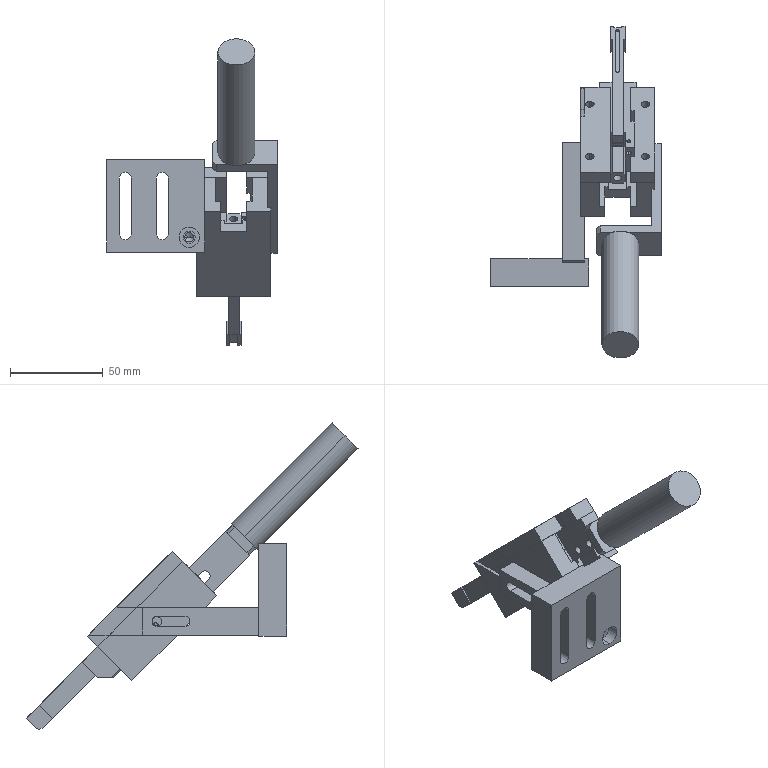Assembly | SolidWorks | mm | 12 component files | 12 solids | 233 faces | box 92 x 179.44 x 165.47 mm | volume 144263 mm3 | plane 140 | cylinder 71 | cone 22 | commonest cylinder face diameters 3 x16 3.3 x8 4.5 x8 4.2 x6 5.5 x5 6.5 x4 5 x4 2 x4
Bill of materials:
Cylinder16X30 | 1 |  | Plain solid round cylinder with flat ends, length roughly 2.5-3 times its diameter.
ZL-10-01BasePlate | 1 |  | Rectangular block or thick plate with two parallel obround through-slots, one round through-hole, and a shallow rectangular notch cut into one top edge.
ZL-10-02SupportPlate | 1 |  | Long rectangular bar with a round hole in one end face, chamfered edges around that end, and an obround through-slot near the opposite end of one side face.
ZL-10-03SlideChannel | 1 |  | Complex rectangular block with a stepped U-shaped slot open at one end, an open slot/channel at the other end, several stepped pockets, shallow side recesses, and four small holes in one face.
ZL-10-04LeftCoverPlate | 1 |  | Thin rectangular bar with two round holes along its length and a shallow rectangular notch or step on one long edge.
ZL-10-05RightCoverPlate | 1 |  | Thin rectangular bar with two round holes and a long shallow step/relief along one long edge between the holes, plus a short edge recess.
ZL-10-06L-shapedBracket | 1 |  | L-shaped angle bracket made from flat strip: the short leg has a round through-hole and chamfered end corners, and the long leg has an obround through-slot.
ZL-10-07Slider | 1 |  | Rectangular plate/block with a stepped open slot at one end, a narrower open slot at the other end, chamfered corners at one end, and several small holes on the faces and edges.
ZL-10-08FloatingJoint | 1 |  | Prismatic bar with a rectangular cross-section and chamfered long edges (octagon-like outline), with a round bore in each end face and a round cross-hole through a side face near one end.
ZL-10-10FloatingJointPin | 2 |  | Long solid round rod/pin with small chamfers at both ends, length roughly 6-7 times its diameter.
ZL3-10-09PressureBlock | 1 |  | Long slender flat strip with one rounded end holding a small round through-hole; near that end there are a small end notch and slightly wider shoulder/lug sections.
Mates:
1. concentric | ZL-10-01BasePlate-1 face at (18.823, -6.251, -17) dir (0, -1, 0) r 3.3 | ZL-10-02SupportPlate-1 face at (18.823, 6.749, -17) dir (0, -1, 0) r 2.5
2. coincident | ZL-10-01BasePlate-1 face at (12.823, 8.749, -25) dir (1, 0, 0) | ZL-10-02SupportPlate-1 face at (12.823, 71.749, -9.5) dir (-1, 0, 0)
3. coincident | ZL-10-01BasePlate-1 face at (24.823, 6.749, -25) dir (0, 1, 0) | ZL-10-02SupportPlate-1 face at (24.823, 6.749, -9.5) dir (0, -1, 0)
4. concentric | ZL-10-02SupportPlate-1 face at (12.823, 63.749, -17) dir (1, 0, 0) r 2.75 | ZL-10-03SlideChannel-1 face at (24.823, 63.749, -17) dir (-1, 0, 0) r 2.5
5. coincident | ZL-10-02SupportPlate-1 face at (24.823, 6.749, -24.5) dir (0, 0, -1) | ZL-10-03SlideChannel-1 face at (24.823, 89.634, -24.5) dir (0, 0, 1)
6. coincident | ZL-10-02SupportPlate-1 face at (24.823, 71.749, -9.5) dir (1, 0, 0) | ZL-10-03SlideChannel-1 face at (24.823, 74.634, -9.5) dir (-1, 0, 0)
7. concentric | ZL-10-03SlideChannel-1 face at (61.323, 52.007, -6.672) dir (1, 0, 0) r 2.1 | ZL-10-06L-shapedBracket-1 face at (31.323, 52.007, -6.672) dir (1, 0, 0) r 2.75
8. coincident | ZL-10-03SlideChannel-1 face at (61.323, 79.584, -46.977) dir (1, 0, 0) | ZL-10-06L-shapedBracket-1 face at (61.323, 13.823, 18.784) dir (-1, 0, 0)
9. coincident | ZL-10-03SlideChannel-1 face at (61.323, 92.312, -34.249) dir (0, -0.7071, -0.7071) | ZL-10-06L-shapedBracket-1 face at (66.323, 26.551, 31.512) dir (0, 0.7071, 0.7071)
10. coincident | ZL-10-03SlideChannel-1 plane at (42.823, 31.501, -3.136) dir (-1, 0, 0) | ZL-10-07Slider-1 plane at (42.823, 56.084, -16.405) dir (-1, 0, 0)
11. coincident | ZL-10-03SlideChannel-1 face at (52.823, 83.119, -43.441) dir (0, 0.7071, 0.7071) | ZL-10-07Slider-1 face at (32.823, 91.439, -51.761) dir (0, -0.7071, -0.7071)
12. concentric | ZL-10-07Slider-1 face at (52.823, 64.569, -19.234) dir (-1, 0, 0) r 1.5 | ZL-10-08FloatingJoint-1 face at (38.823, 64.569, -19.234) dir (1, 0, 0) r 1.5
13. coincident | ZL-10-07Slider-1 plane at (42.823, 56.084, -16.405) dir (-1, 0, 0) | ZL-10-08FloatingJoint-1 plane at (42.823, 52.548, -7.213) dir (1, 0, 0)
14. coincident | ZL-10-07Slider-1 face at (45.823, 97.096, -46.104) dir (0, 0.7071, 0.7071) | ZL-10-08FloatingJoint-1 face at (38.823, 69.519, -18.527) dir (0, 0.7071, 0.7071)
15. coincident | ZL-10-03SlideChannel-1 face at (22.823, 95.847, -30.713) dir (0, 0.7071, 0.7071) | ZL-10-04LeftCoverPlate-1 face at (22.823, 95.847, -30.713) dir (0, -0.7071, -0.7071)
16. coincident | ZL-10-03SlideChannel-1 face at (62.823, 95.847, -30.713) dir (0, 0.7071, 0.7071) | ZL-10-05RightCoverPlate-1 face at (49.823, 95.847, -30.713) dir (0, -0.7071, -0.7071)
17. concentric | ZL-10-07Slider-1 face at (32.823, 75.883, -17.82) dir (1, 0, 0) r 1.5 | ZL3-10-09PressureBlock-1 face at (38.823, 75.883, -17.82) dir (1, 0, 0) r 1.5
18. coincident | ZL-10-07Slider-1 plane at (42.823, 56.084, -16.405) dir (-1, 0, 0) | ZL3-10-09PressureBlock-1 plane at (42.823, 75.175, -10.041) dir (1, 0, 0)
19. coincident | ZL-10-07Slider-1 face at (45.823, 97.096, -46.104) dir (0, 0.7071, 0.7071) | ZL3-10-09PressureBlock-1 face at (45.823, 68.104, -17.112) dir (0, -0.7071, -0.7071)
20. concentric | ZL-10-07Slider-1 face at (52.823, 64.569, -19.234) dir (-1, 0, 0) r 1.5 | ZL-10-10FloatingJointPin-1 face at (32.823, 64.569, -19.234) dir (1, 0, 0) r 1.5
21. coincident | ZL-10-07Slider-1 face at (52.823, 91.439, -51.761) dir (1, 0, 0) | ZL-10-10FloatingJointPin-1 face at (52.823, 64.569, -19.234) dir (1, 0, 0)
22. concentric | ZL-10-07Slider-1 face at (32.823, 75.883, -17.82) dir (1, 0, 0) r 1.5 | ZL-10-10FloatingJointPin-2 face at (52.823, 75.883, -17.82) dir (-1, 0, 0) r 1.5
23. coincident | ZL-10-07Slider-1 face at (52.823, 91.439, -51.761) dir (1, 0, 0) | ZL-10-10FloatingJointPin-2 face at (52.823, 75.883, -17.82) dir (1, 0, 0)
24. concentric | ZL-10-03SlideChannel-1 face at (27.823, 58.371, 6.763) dir (0, 0.7071, 0.7071) r 1.65 | ZL-10-04LeftCoverPlate-1 face at (27.823, 58.371, 6.763) dir (0, 0.7071, 0.7071) r 2.25
25. concentric | ZL-10-03SlideChannel-1 face at (27.823, 86.655, -21.521) dir (0, 0.7071, 0.7071) r 1.65 | ZL-10-04LeftCoverPlate-1 face at (27.823, 86.655, -21.521) dir (0, 0.7071, 0.7071) r 2.25
26. concentric | ZL-10-03SlideChannel-1 face at (57.823, 86.655, -21.521) dir (0, 0.7071, 0.7071) r 1.65 | ZL-10-05RightCoverPlate-1 face at (57.823, 86.655, -21.521) dir (0, 0.7071, 0.7071) r 2.25
27. concentric | ZL-10-03SlideChannel-1 face at (57.823, 58.371, 6.763) dir (0, 0.7071, 0.7071) r 1.65 | ZL-10-05RightCoverPlate-1 face at (57.823, 58.371, 6.763) dir (0, 0.7071, 0.7071) r 2.25
28. concentric | ZL-10-06L-shapedBracket-1 face at (44.323, 66.149, -20.814) dir (0, -0.7071, 0.7071) r 5.25 | Cylinder16X30-1 face at (44.323, -37.796, 83.131) dir (0, 0.7071, -0.7071) r 10
29. coincident | ZL-10-06L-shapedBracket-1 face at (66.323, 10.287, 22.32) dir (0, -0.7071, 0.7071) | Cylinder16X30-1 face at (44.323, 16.651, 28.684) dir (0, 0.7071, -0.7071)
30. coincident | ZL-10-06L-shapedBracket-1 plane at (66.323, 16.651, 28.684) dir (0, -0.7071, -0.7071) | Cylinder16X30-1 plane at (44.323, 16.651, 28.684) dir (0, 0.7071, 0.7071)